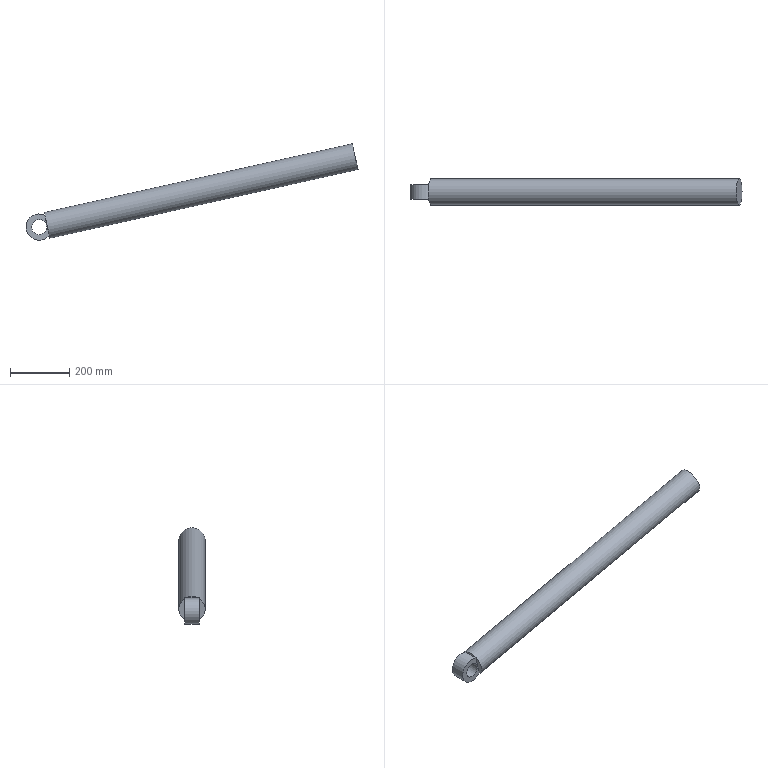Component | NX | LARGE_ARM_EXT_ROD | 1 solid | 7 faces | volume 6778037 mm3 | plane 4 | cylinder 3 | commonest cylinder face diameters 88.9 x2 50.8 x1